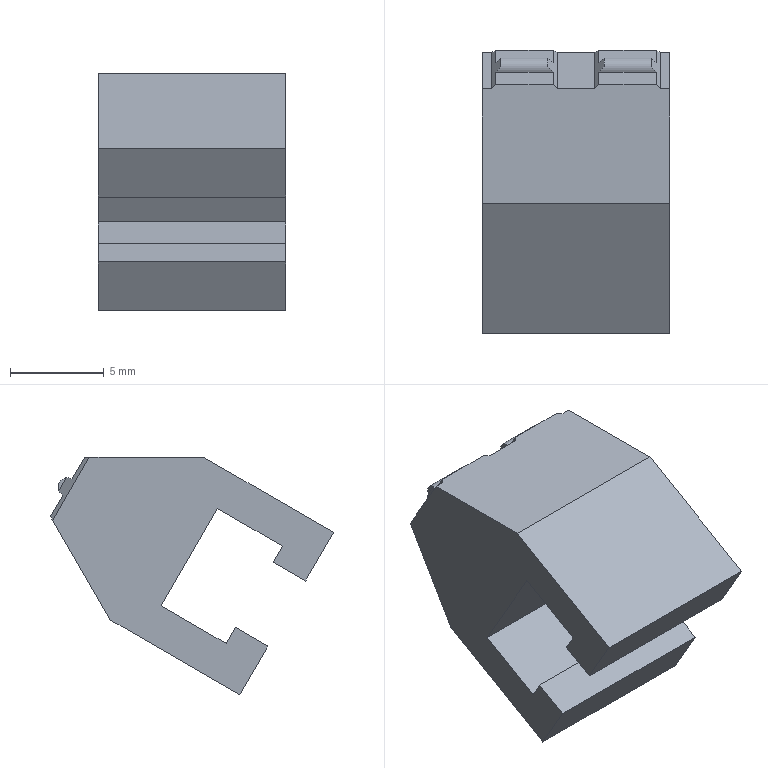Component | NX | CLAMPING_BLOCK | 1 solid | 32 faces | volume 855 mm3 | plane 30 | cylinder 2 | commonest cylinder face diameters 1 x2